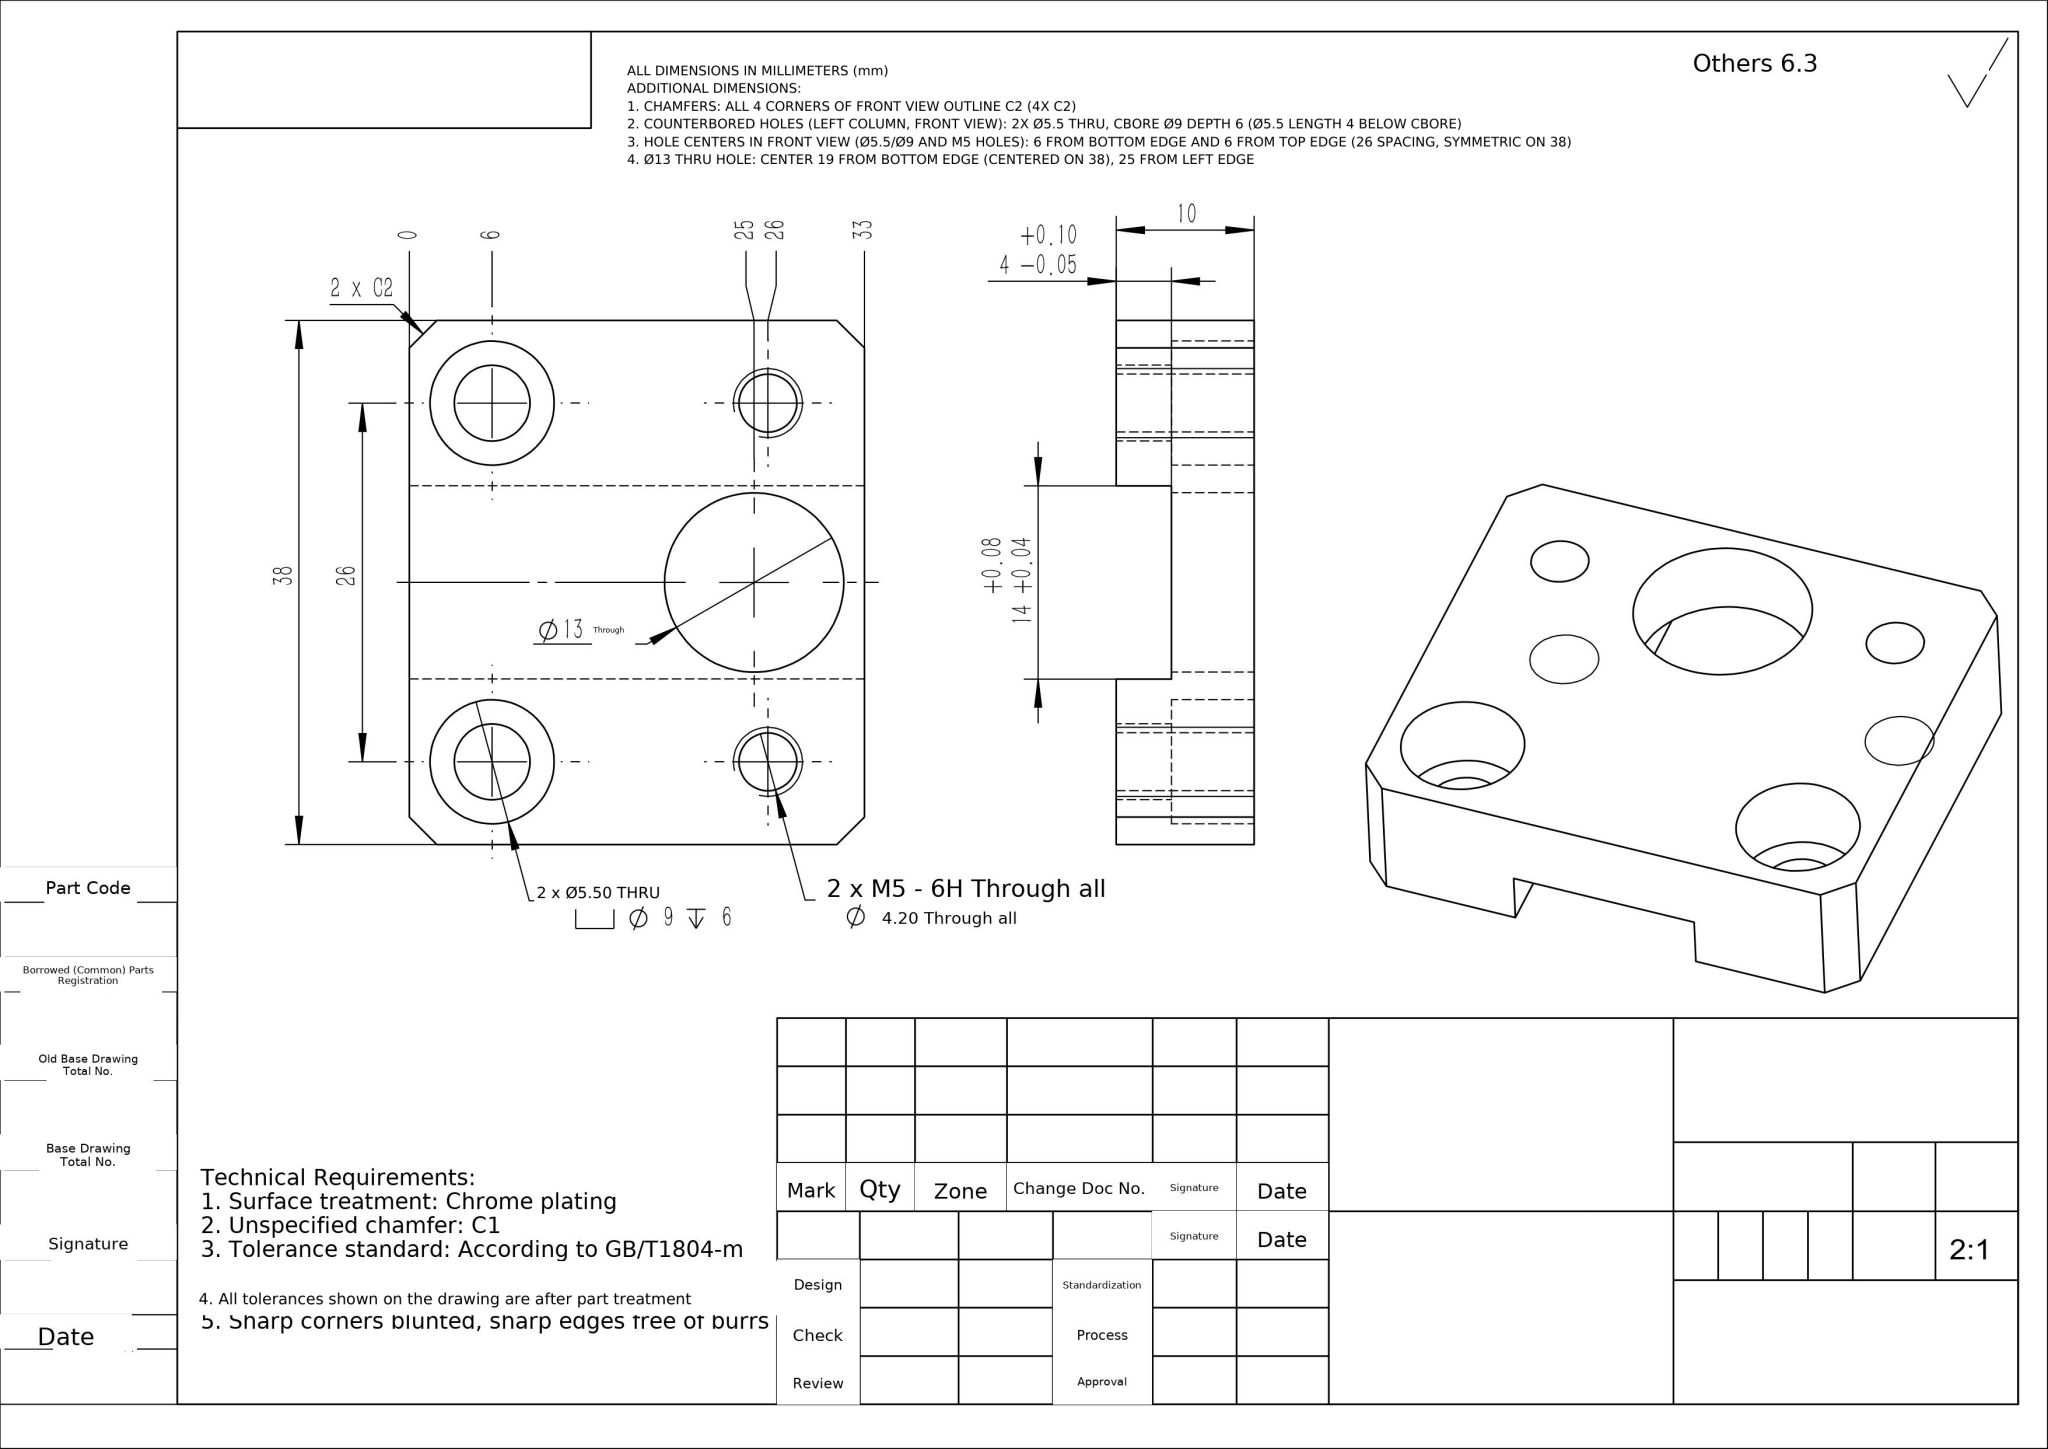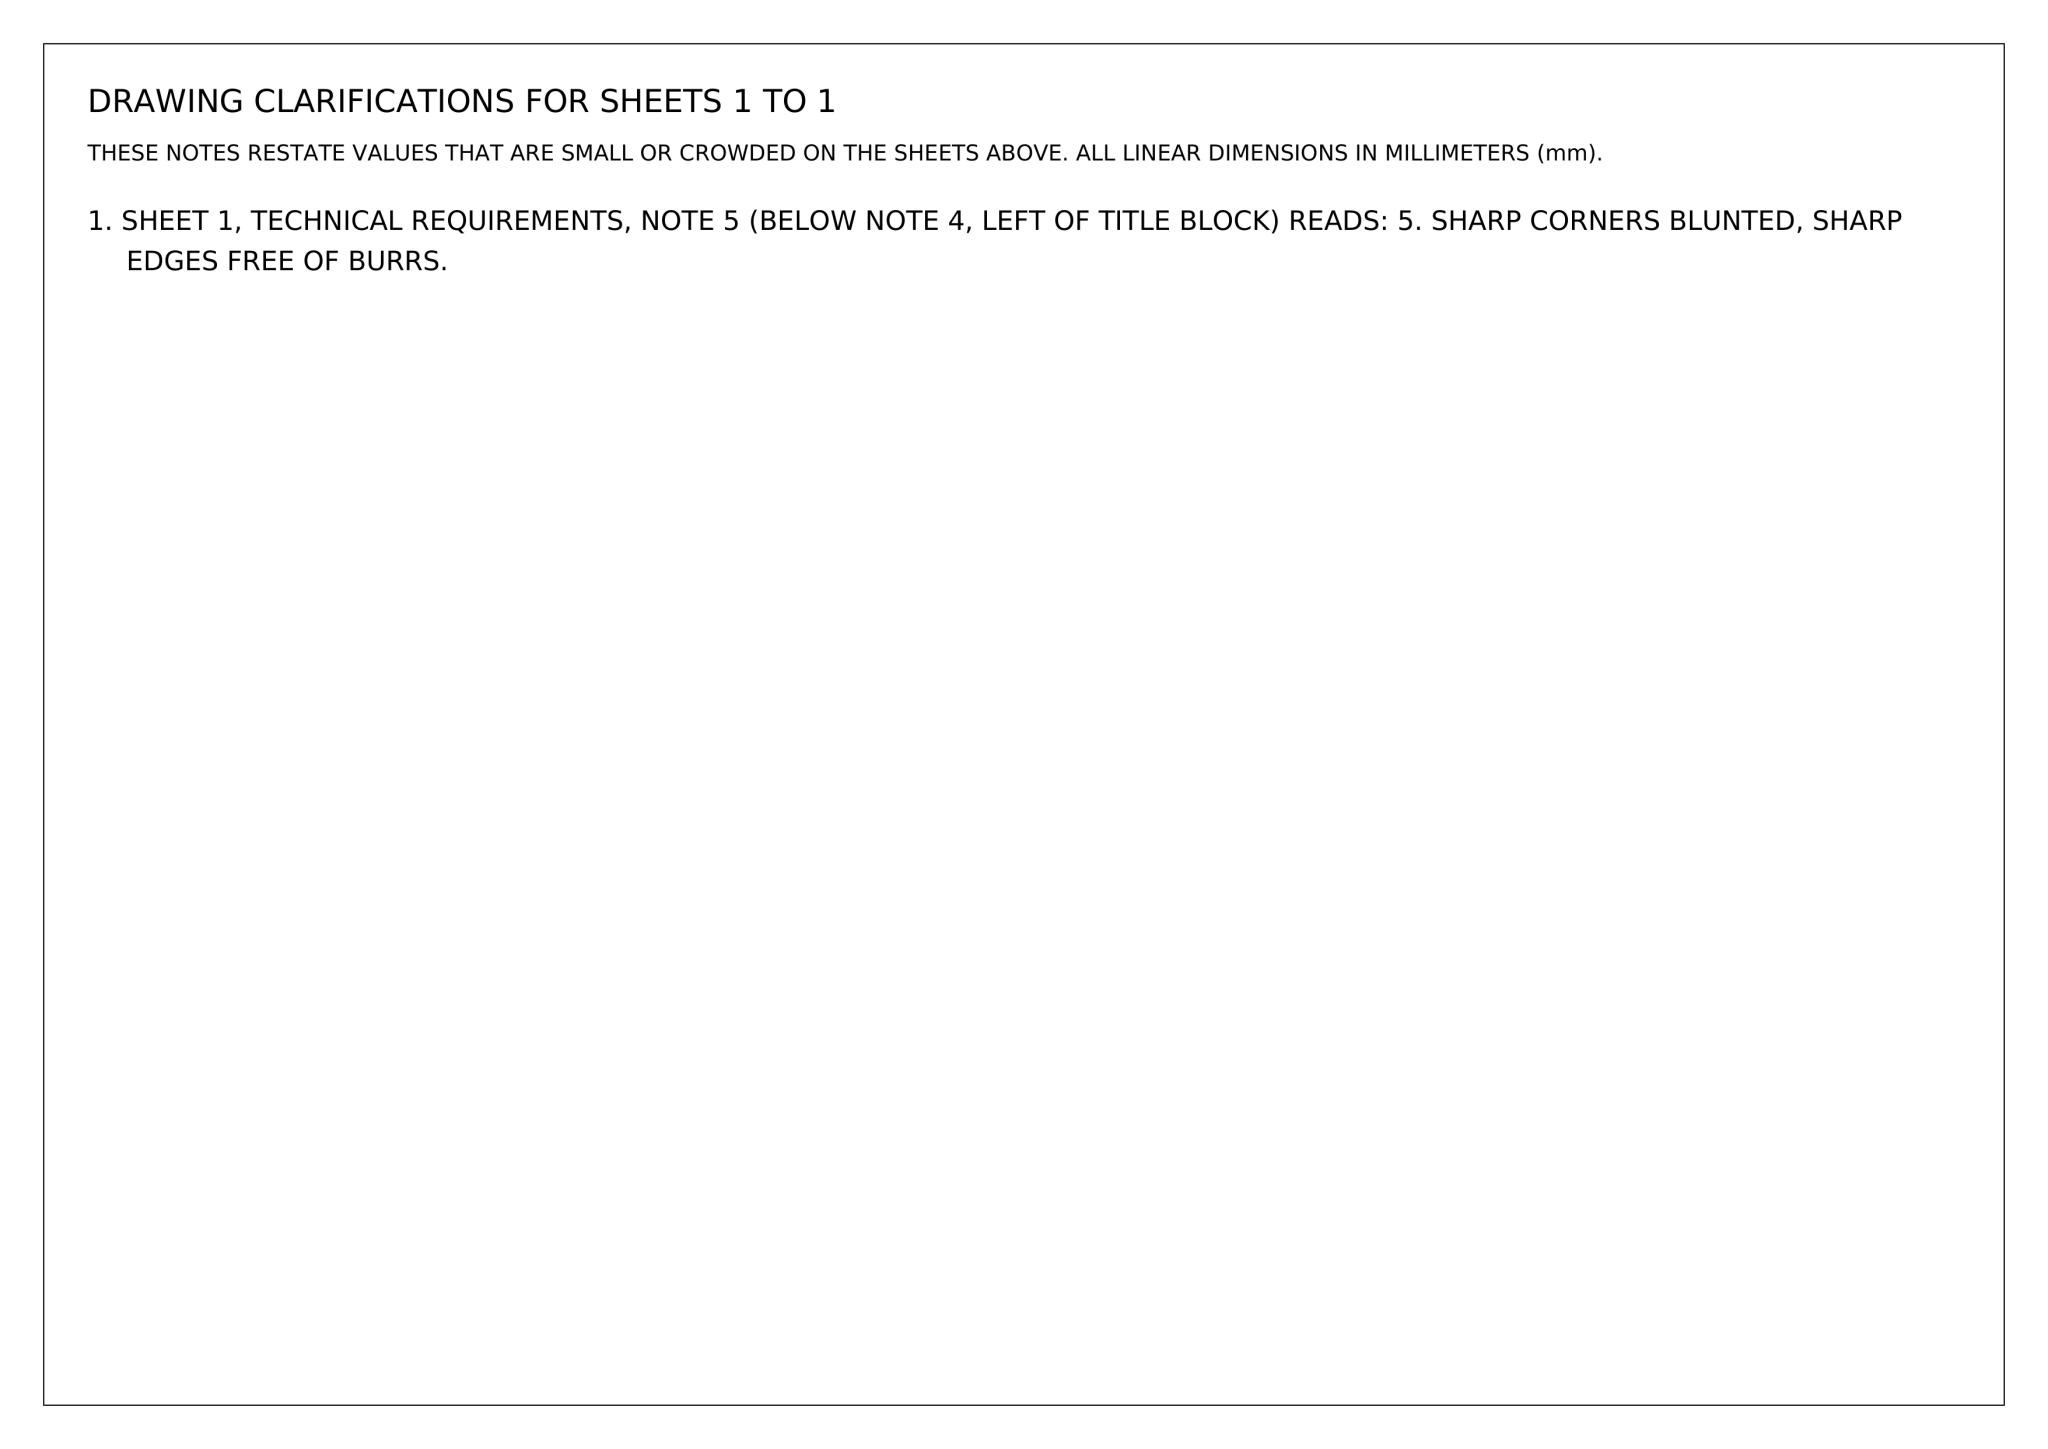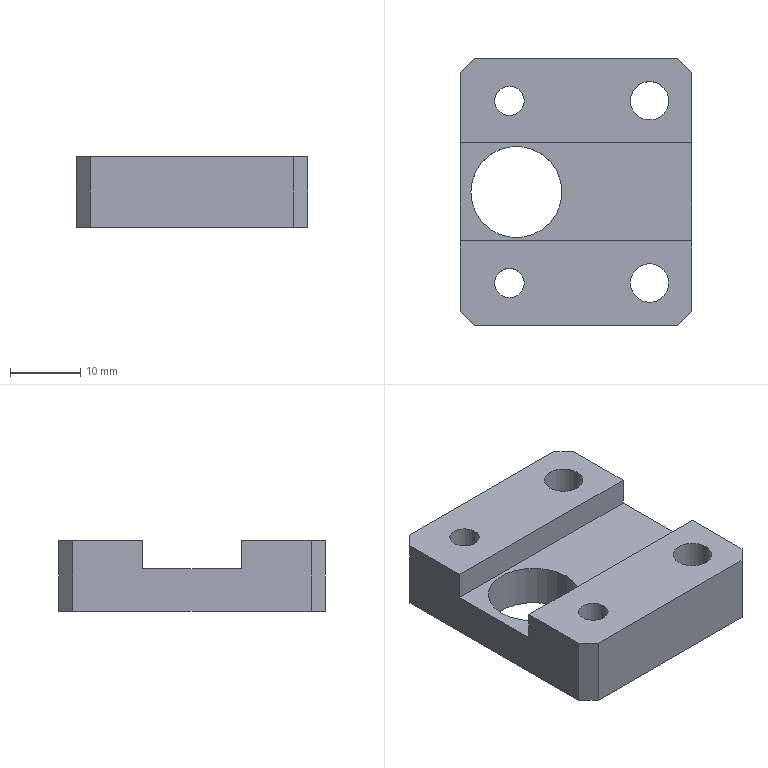Part | NX | mm | 1 solid | 30 faces | box 33 x 38 x 10 mm | volume 8585 mm3 | plane 16 | cylinder 14 | commonest cylinder face diameters 5.5 x4 9 x4 4.2 x4 13 x2